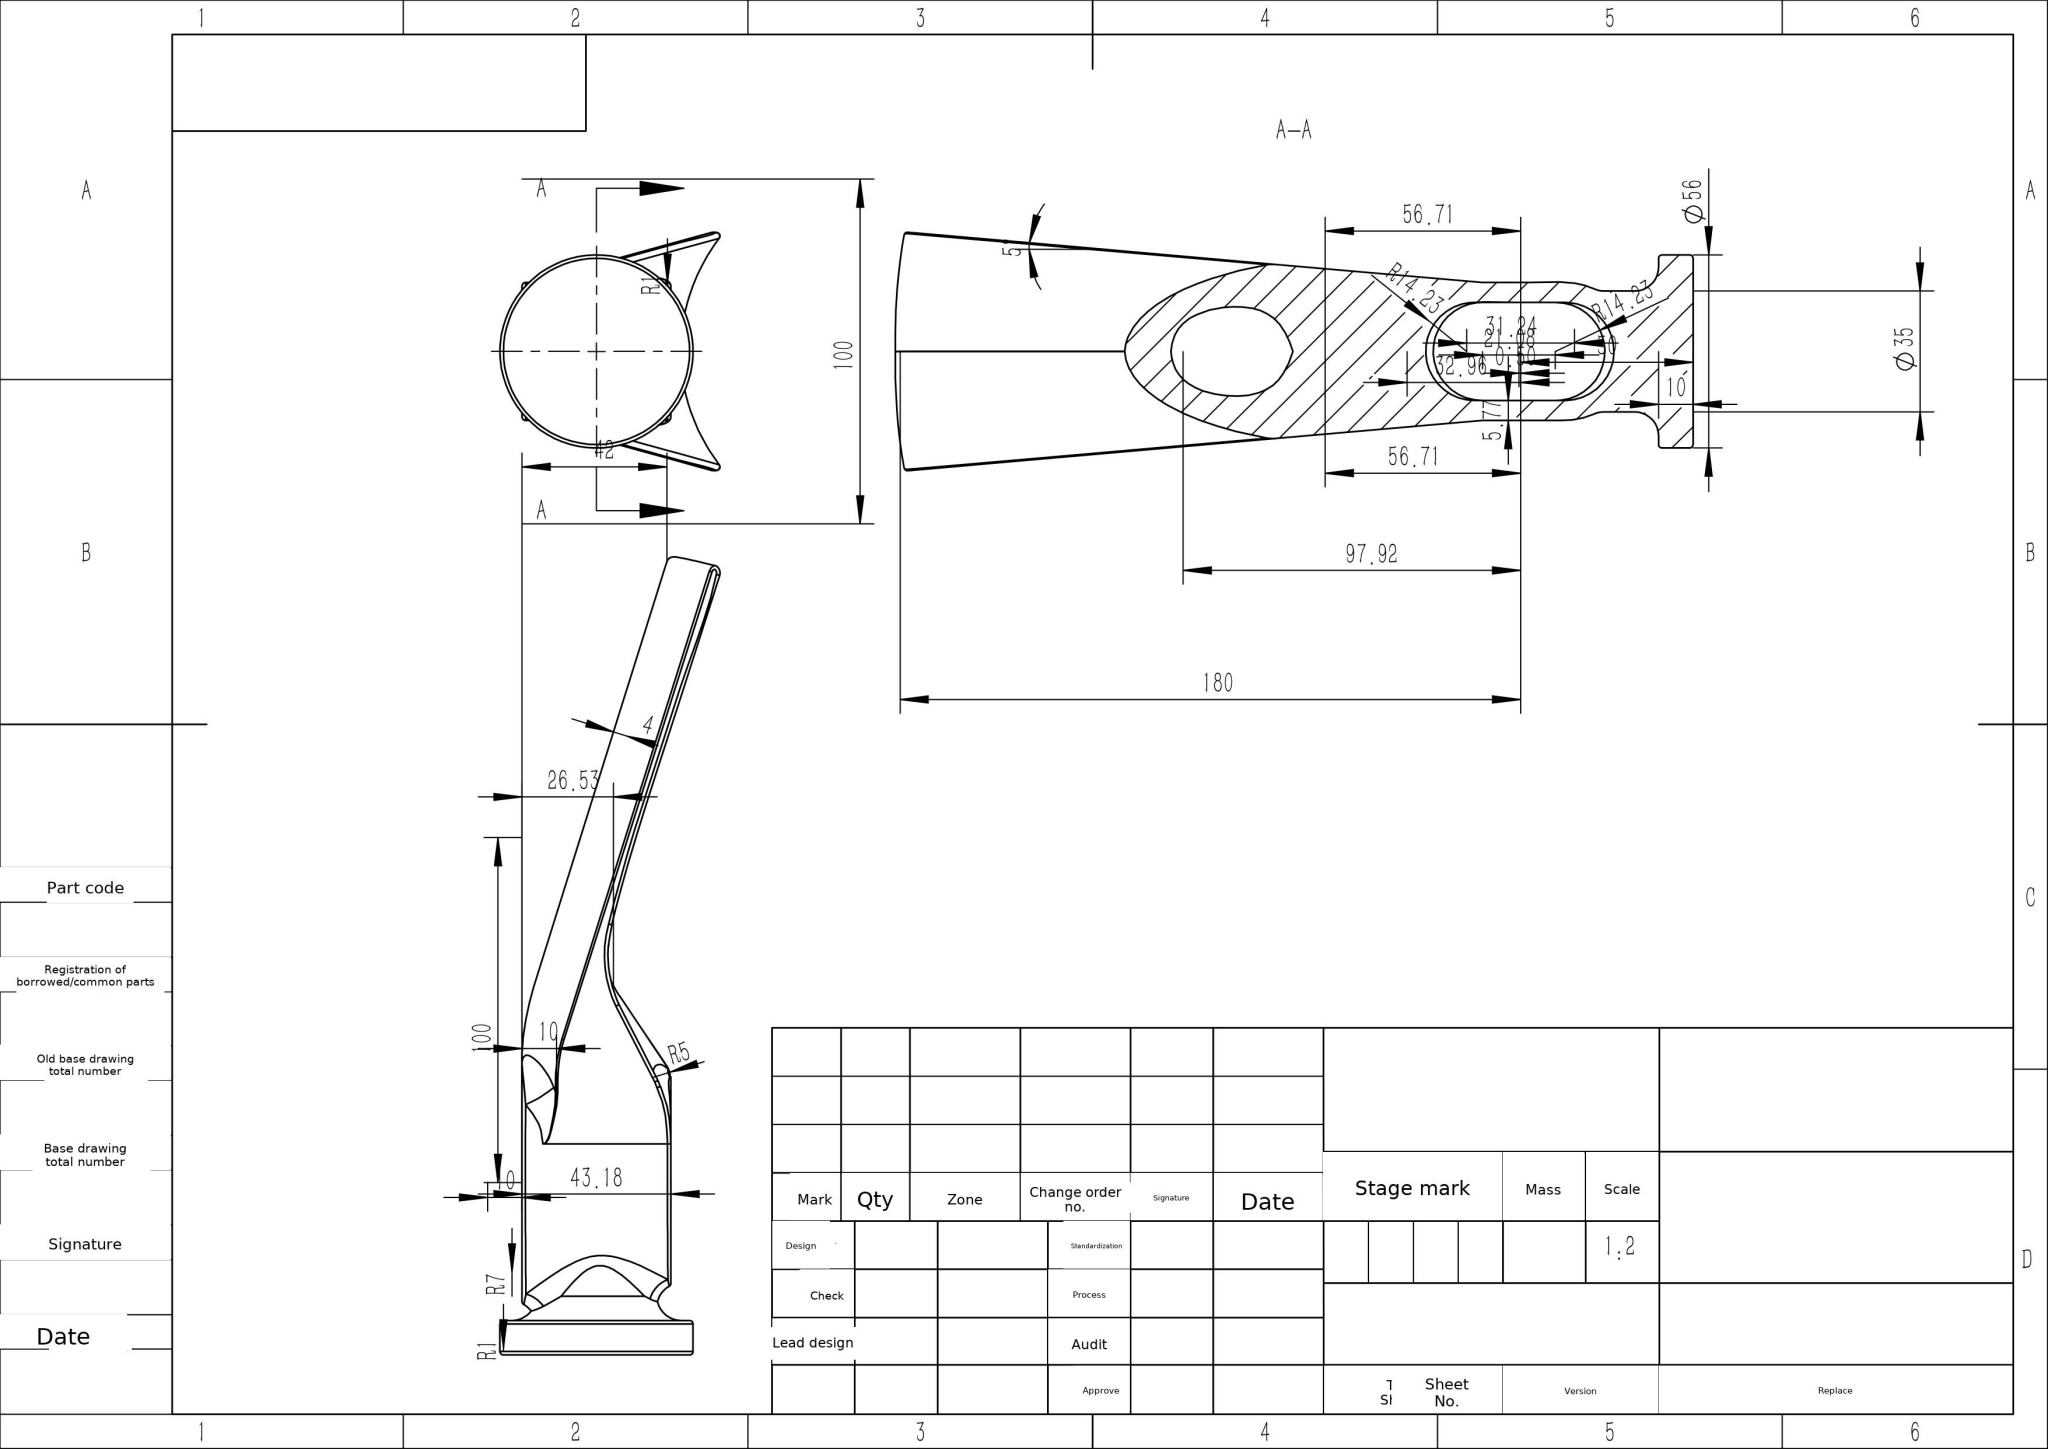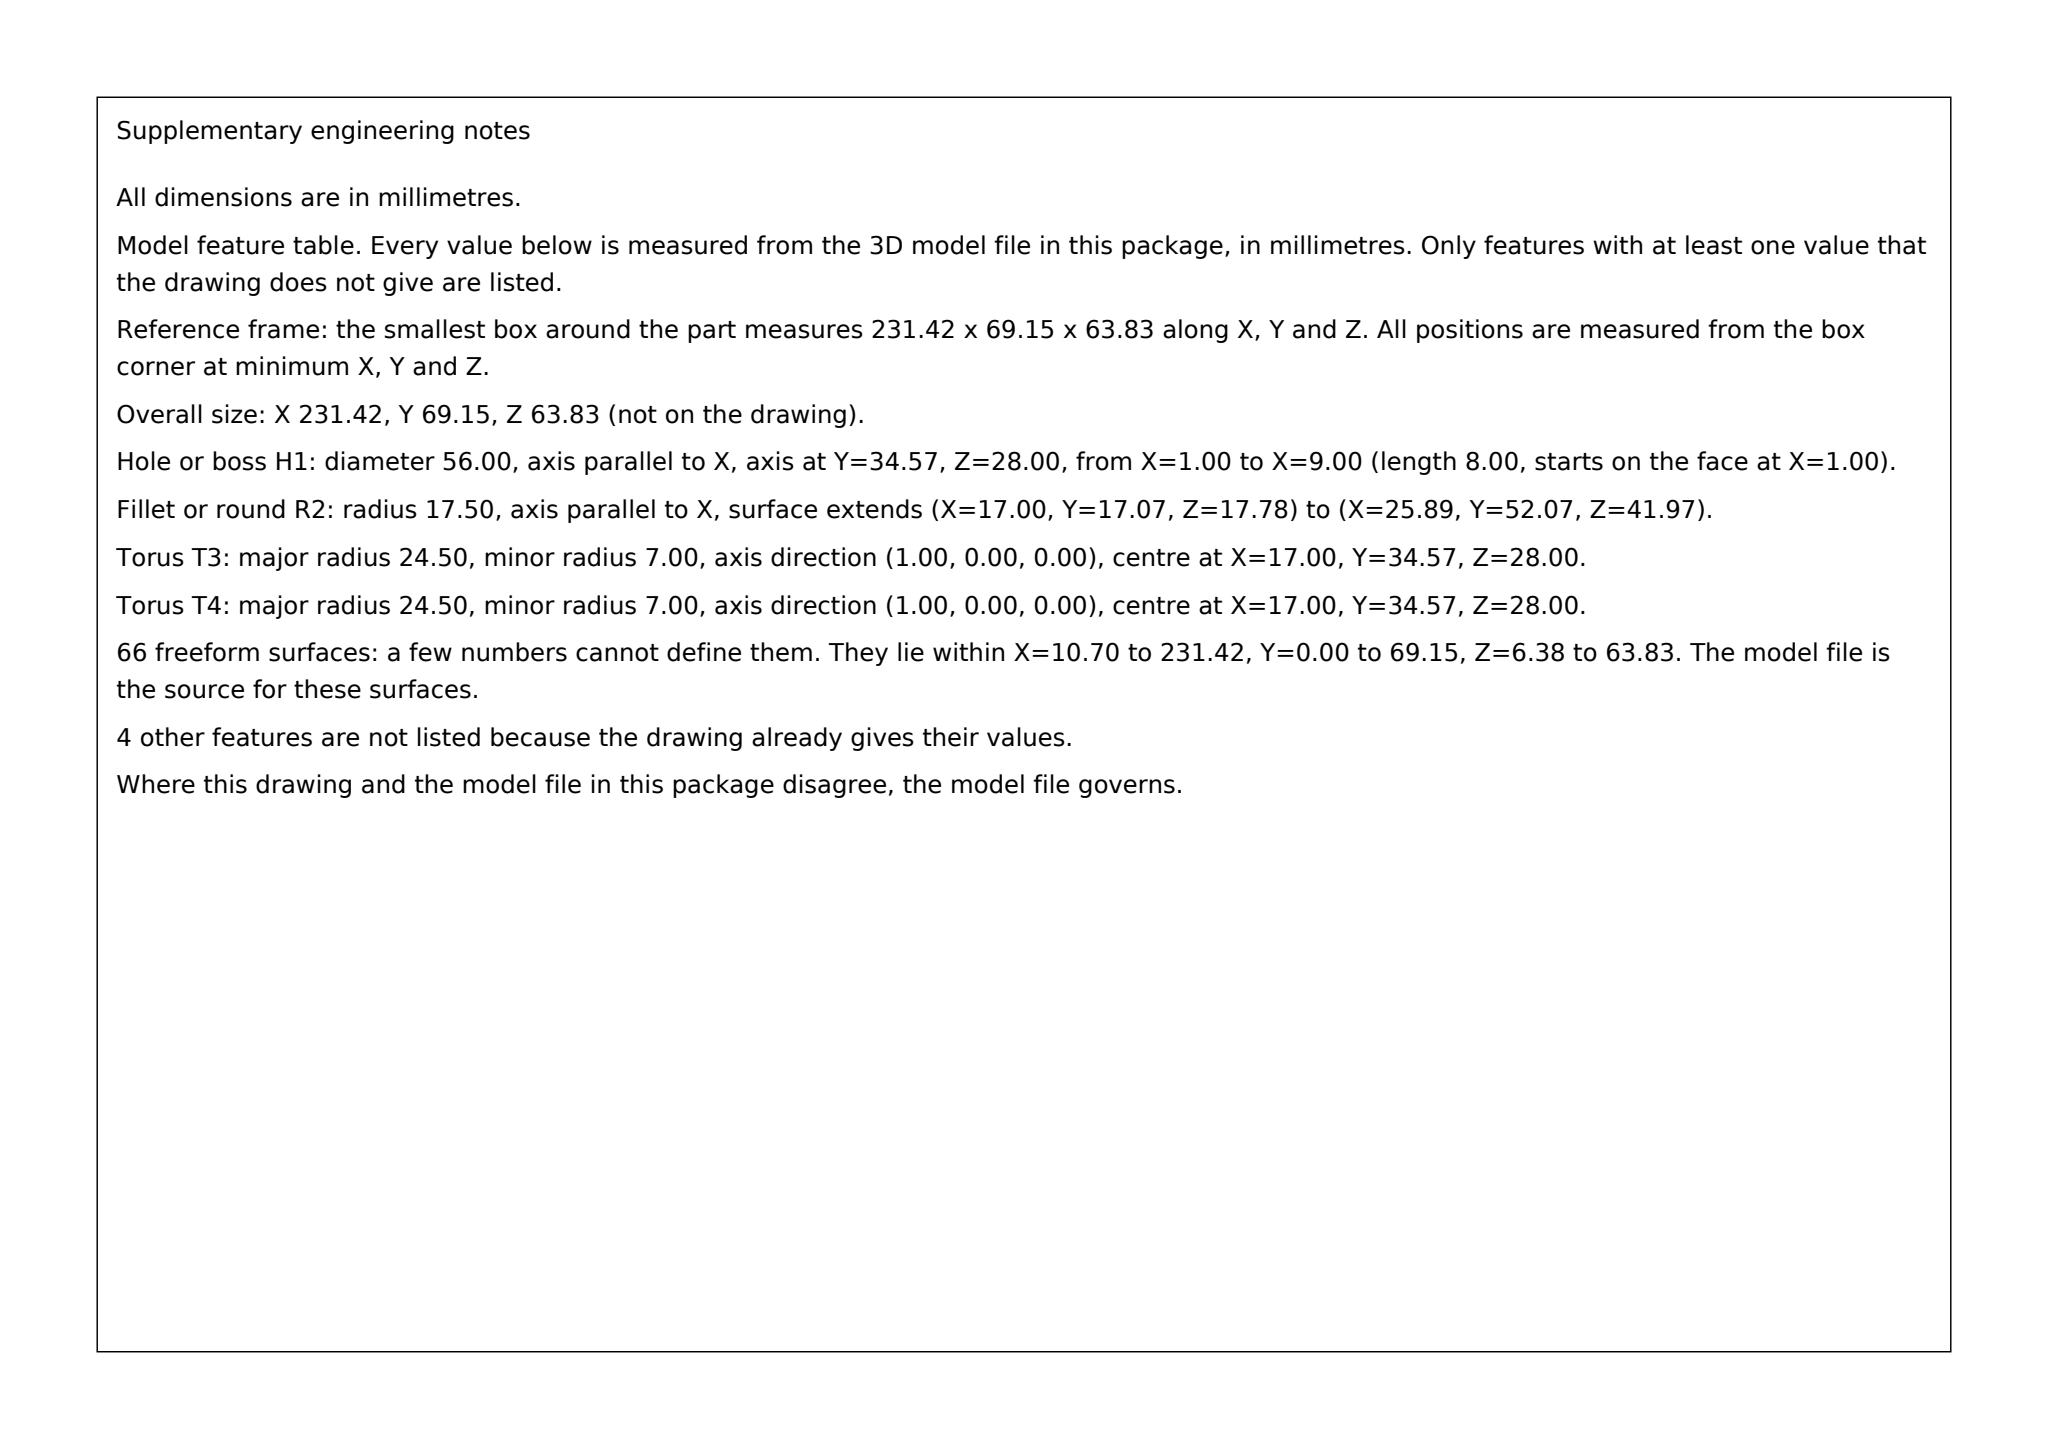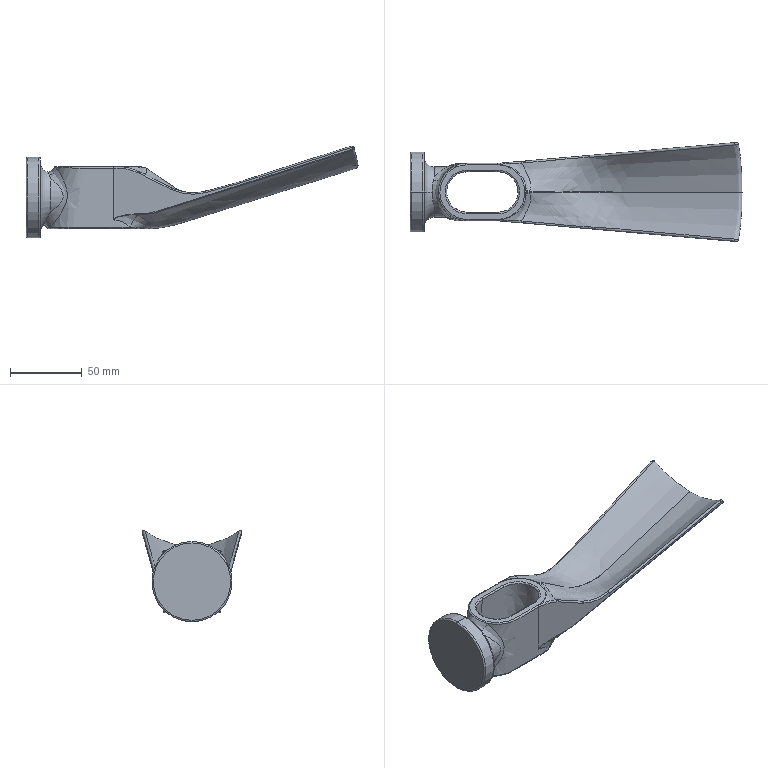Part | SolidWorks | mm | 1 solid | 82 faces | box 231.42 x 69.15 x 63.83 mm | volume 156000 mm3 | spline 66 | torus 6 | plane 6 | cylinder 4 | commonest cylinder face diameters 56 x2 35 x2